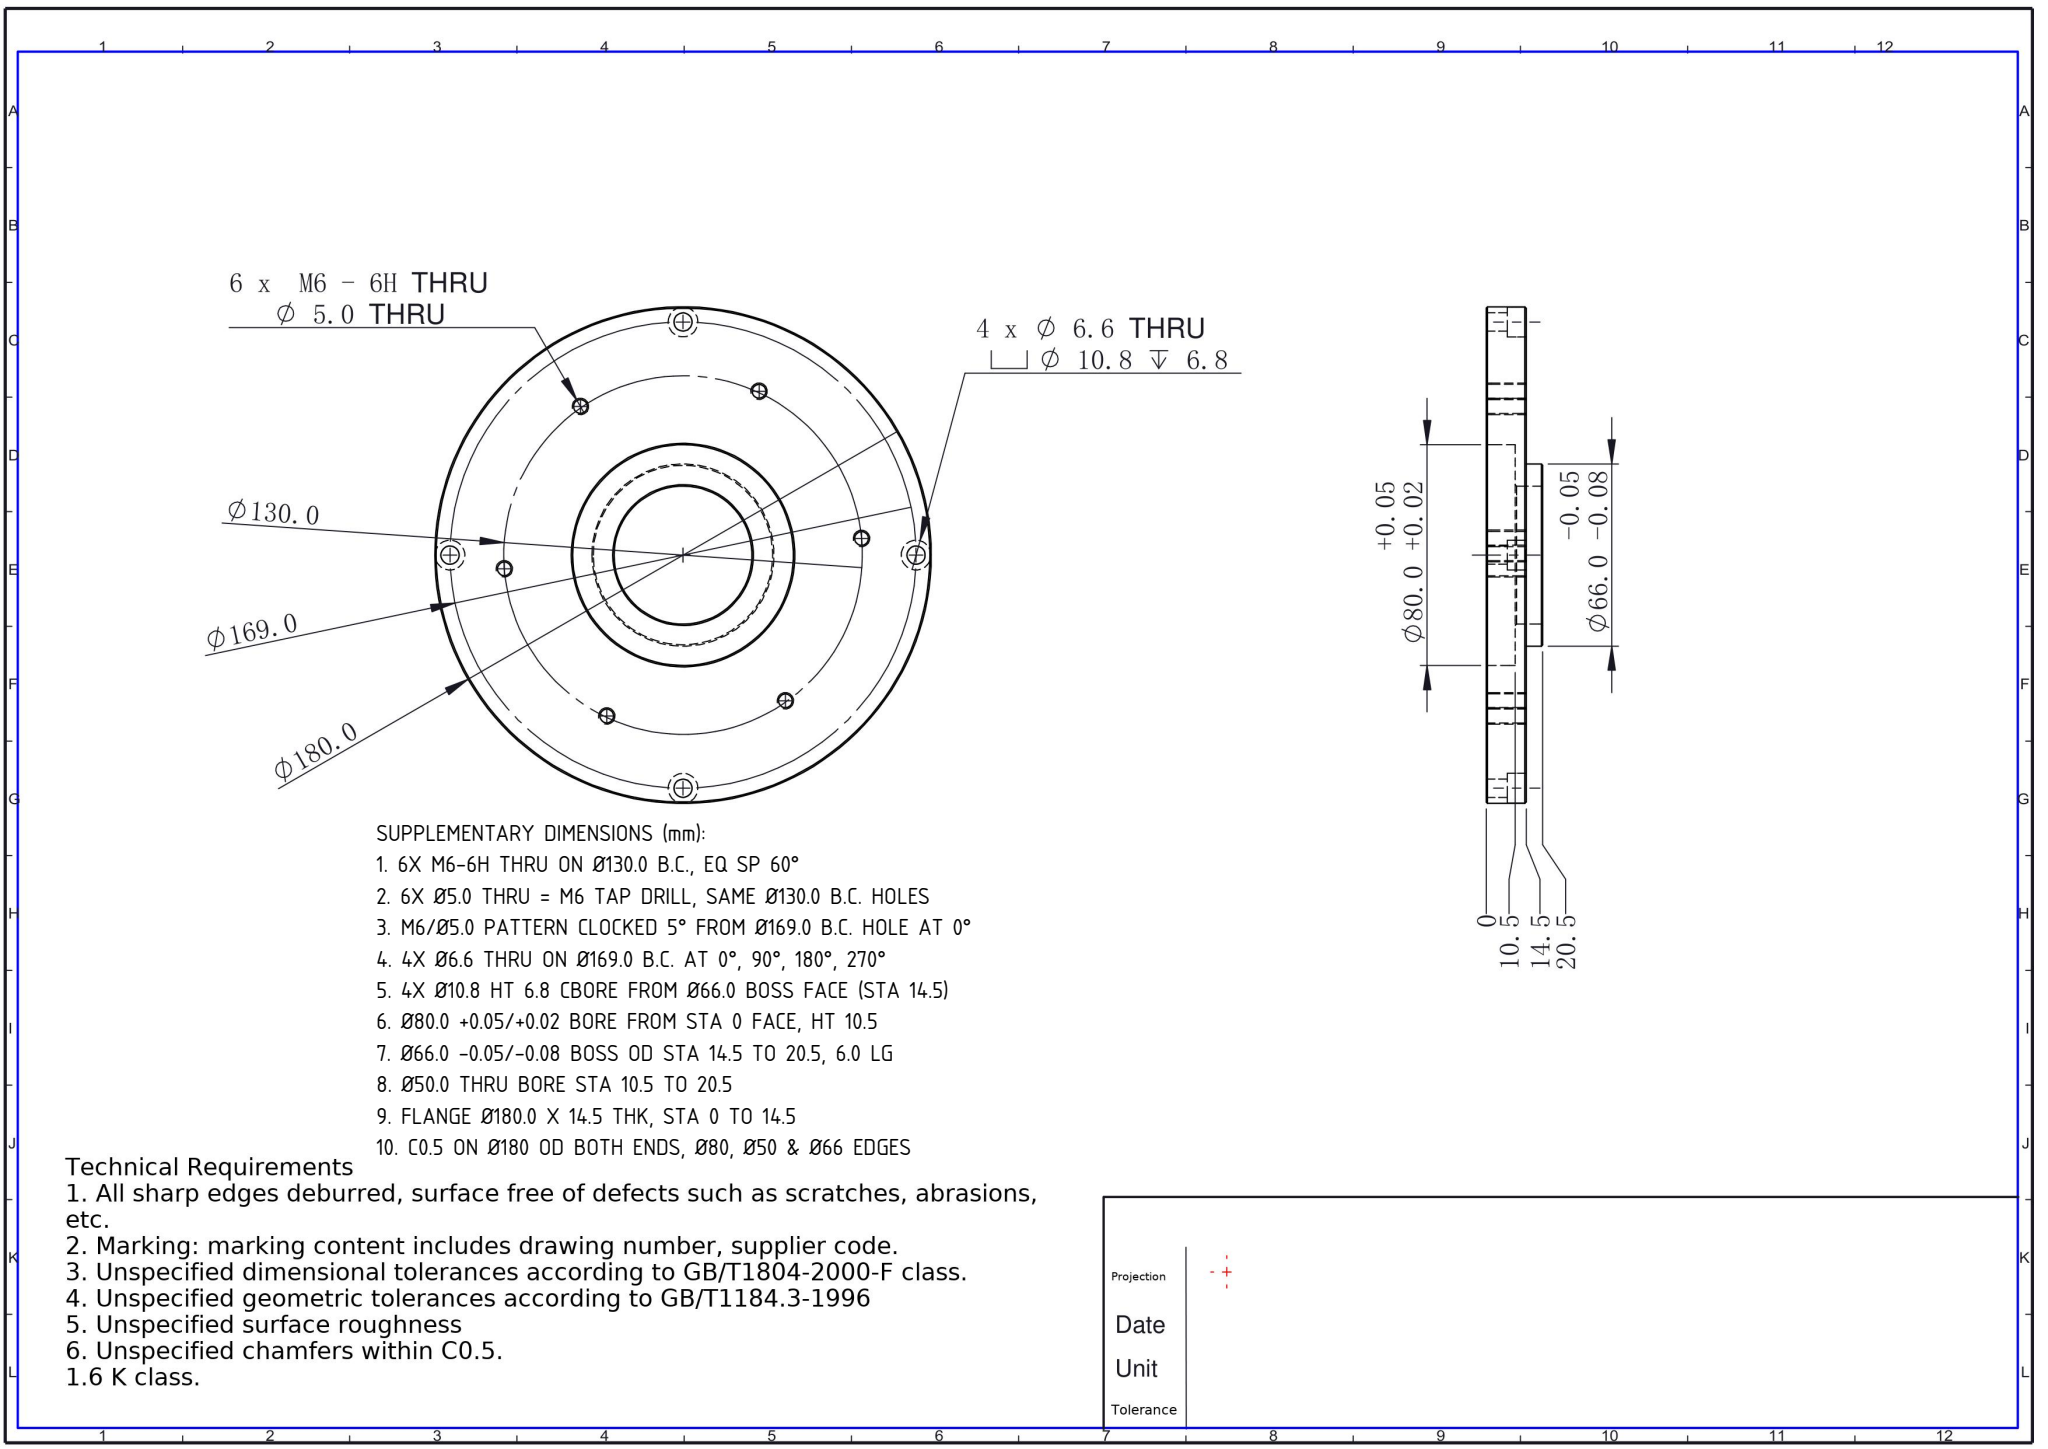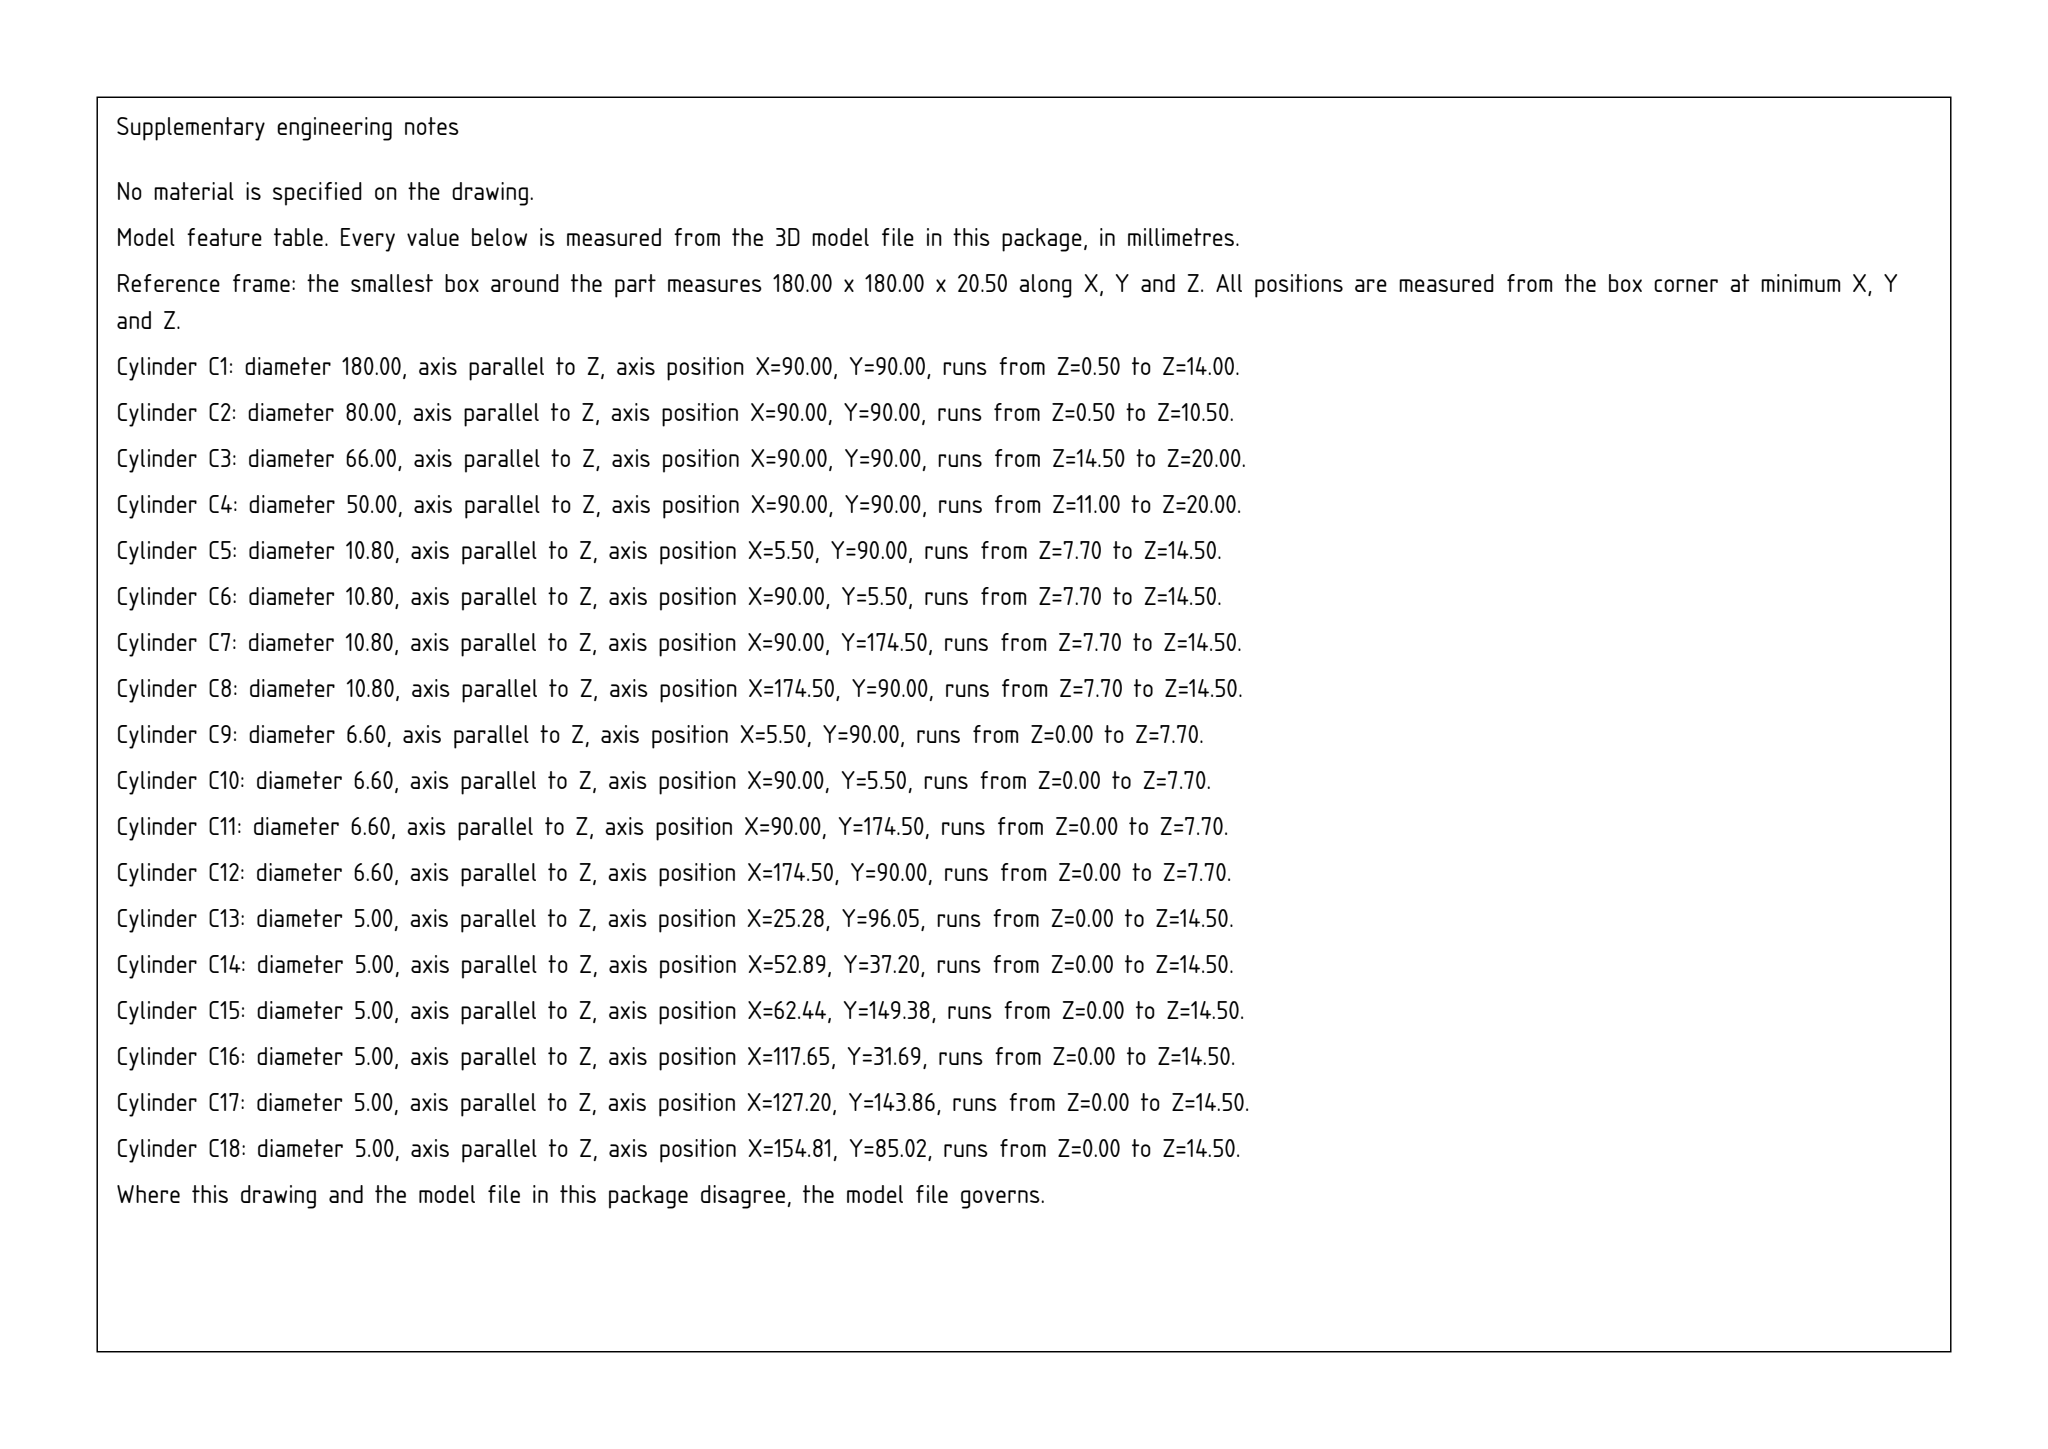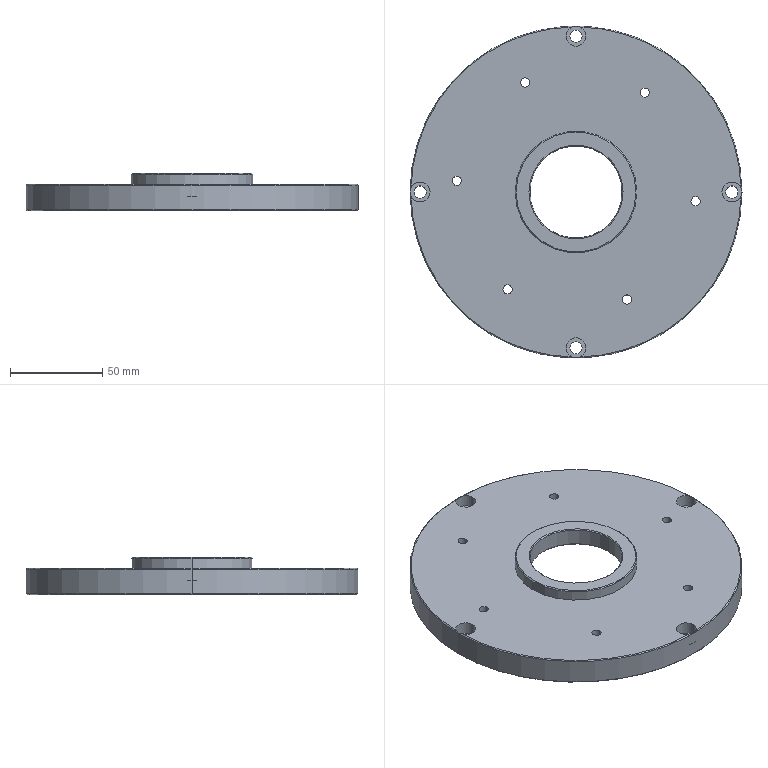Part | SolidWorks | mm | 1 solid | 56 faces | box 180 x 180 x 20.5 mm | volume 311603 mm3 | cylinder 36 | cone 12 | plane 8 | commonest cylinder face diameters 5 x12 10.8 x8 6.6 x8 66 x2 50 x2 180 x2 80 x2